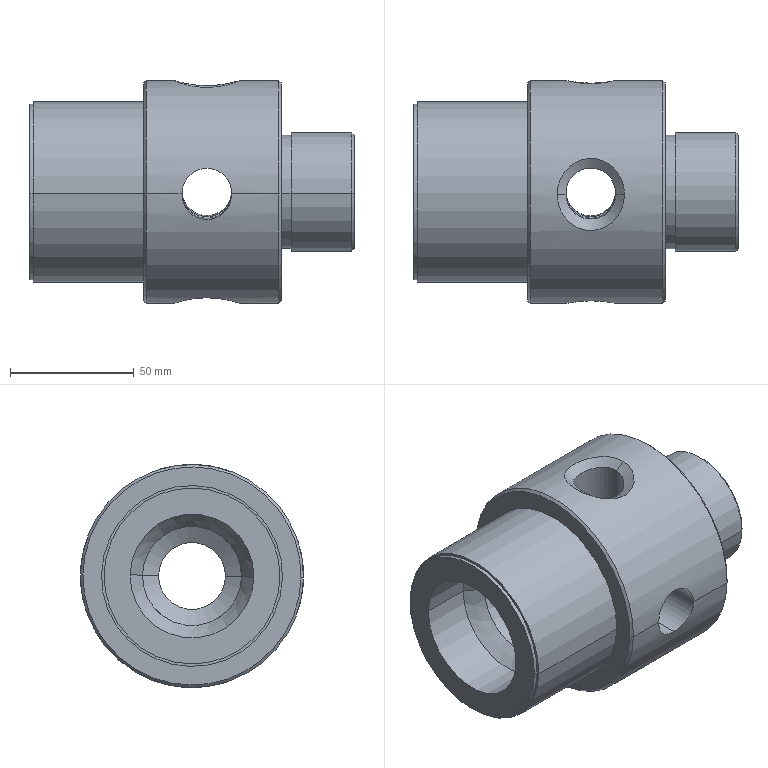Component | SolidWorks | 216InnerTubeAssembly-1_Adapter-1 | 1 solid | 58 faces | volume 412344 mm3 | cylinder 36 | cone 12 | plane 6 | spline 4 | commonest cylinder face diameters 20 x20 46 x2 48 x2 27 x2 40 x2 50 x2 71 x2 73 x2 | material Alloy Steel